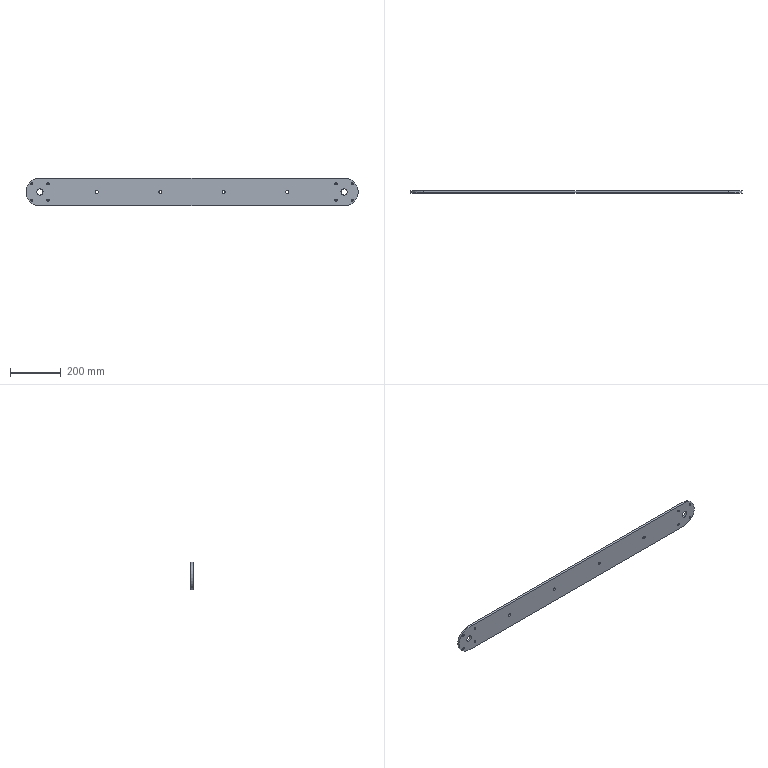Component | NX | 131_MOUNT_PLATE_BASE | 1 solid | 20 faces | volume 1116922 mm3 | cylinder 16 | plane 4 | commonest cylinder face diameters 8.5 x8 12 x4 110 x2 25 x2